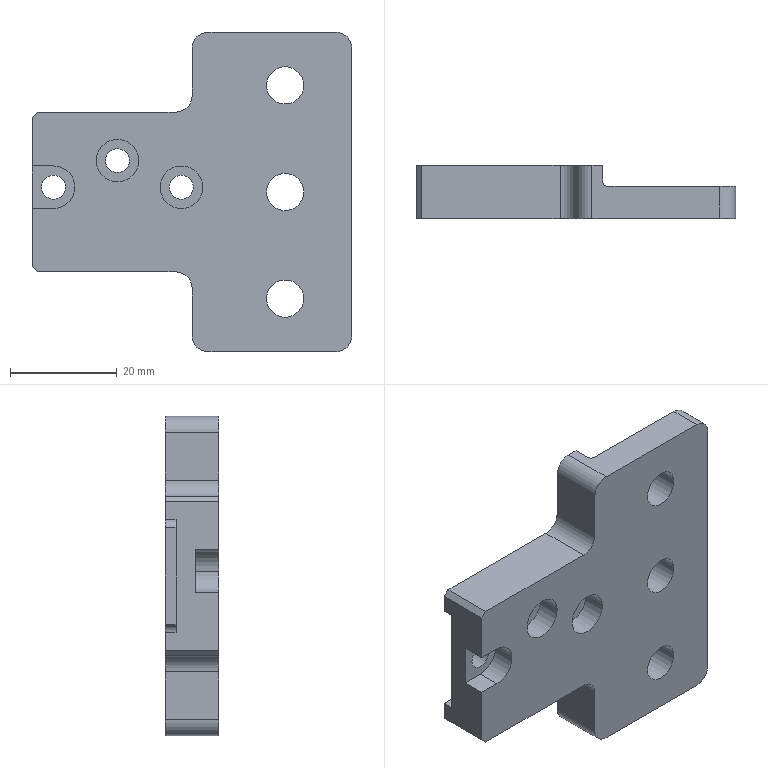Component | SolidWorks | SAWH02-03342A0SuctionCupMountingBase(RightPart)-2 | 1 solid | 50 faces | volume 18043 mm3 | cylinder 27 | plane 23 | commonest cylinder face diameters 4.5 x6 8 x6 7 x6 6 x6 3 x2 2 x1 | material 6061